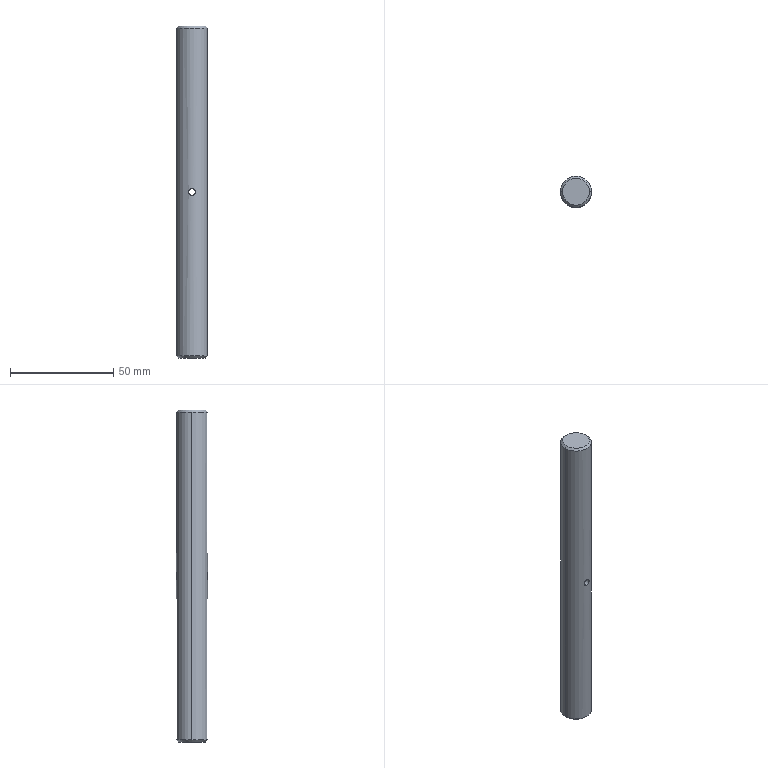Component | SolidWorks | Roller-01-2-1_XT-1-08-2-1 | 1 solid | 10 faces | box 15 x 15 x 160.5 mm | volume 28190 mm3 | cylinder 4 | cone 4 | plane 2 | commonest cylinder face diameters 3.3 x2 15 x2
build123d program:
from build123d import *

# Parameters (mm, degrees)
SKETCH1_R           = 7.5
BOSS_EXTRUDE1_DEPTH = 160.5
CHAMFER1_SIZE       = 1
M4_TAPPED_HOLE1_D   = 3.3


with BuildPart() as part:
    # Sketch1 → Boss-Extrude1 (new body)
    with BuildSketch(Plane.XY):
        Circle(SKETCH1_R)
    extrude(amount=BOSS_EXTRUDE1_DEPTH)

    # Chamfer1
    chamfer1_edges = [part.edges().sort_by_distance(p)[0] for p in [
        (-7.5, 0, 0),
        (-7.5, 0, 160.5),
    ]]
    chamfer(chamfer1_edges, length=CHAMFER1_SIZE)

    # M4 Tapped Hole1 (through all)
    with Locations(Plane(origin=(0, 8.5, 0), x_dir=(1, 0, 0), z_dir=(0, 1, 0))):
        with Locations((0, -80.25)):
            Hole(M4_TAPPED_HOLE1_D / 2)


solid = part.part

# Placed as in the assembly
solid = solid.moved(Location((444.783, 71.385, -153), (0, 0, 0)))
STEP:
#1=CARTESIAN_POINT('',(17.511,2.515,-2.929));
#2=VERTEX_POINT('',#1);
#3=CARTESIAN_POINT('',(17.511,2.515,-2.799));
#4=VERTEX_POINT('',#3);
#5=CARTESIAN_POINT('',(17.511,2.515,-2.929));
#6=CARTESIAN_POINT('',(17.503,2.515,-2.929));
#7=CARTESIAN_POINT('',(17.494,2.516,-2.927));
#8=CARTESIAN_POINT('',(17.482,2.517,-2.923));
#9=CARTESIAN_POINT('',(17.479,2.517,-2.921));
#10=CARTESIAN_POINT('',(17.471,2.518,-2.916));
#11=CARTESIAN_POINT('',(17.468,2.518,-2.913));
#12=CARTESIAN_POINT('',(17.462,2.519,-2.907));
#13=CARTESIAN_POINT('',(17.46,2.52,-2.904));
#14=CARTESIAN_POINT('',(17.455,2.521,-2.897));
#15=CARTESIAN_POINT('',(17.453,2.521,-2.893));
#16=CARTESIAN_POINT('',(17.448,2.522,-2.881));
#17=CARTESIAN_POINT('',(17.446,2.522,-2.873));
#18=CARTESIAN_POINT('',(17.446,2.522,-2.86));
#19=CARTESIAN_POINT('',(17.447,2.522,-2.856));
#20=CARTESIAN_POINT('',(17.448,2.522,-2.847));
#21=CARTESIAN_POINT('',(17.45,2.522,-2.843));
#22=CARTESIAN_POINT('',(17.454,2.521,-2.831));
#23=CARTESIAN_POINT('',(17.459,2.52,-2.824));
#24=CARTESIAN_POINT('',(17.471,2.518,-2.812));
#25=CARTESIAN_POINT('',(17.478,2.517,-2.807));
#26=CARTESIAN_POINT('',(17.49,2.516,-2.803));
#27=CARTESIAN_POINT('',(17.494,2.516,-2.801));
#28=CARTESIAN_POINT('',(17.503,2.515,-2.8));
#29=CARTESIAN_POINT('',(17.507,2.515,-2.799));
#30=CARTESIAN_POINT('',(17.511,2.515,-2.799));
#31=B_SPLINE_CURVE_WITH_KNOTS('',3,(#5,#6,#7,#8,#9,#10,#11,#12,#13,#14,#15,#16,#17,#18,#19,#20,#21,#22,#23,#24,#25,#26,#27,#28,#29,#30),.UNSPECIFIED.,.F.,.F.,(4,2,2,2,2,2,2,2,2,2,2,2,4),(0.005175,0.005821,0.006144,0.006468,0.006791,0.007114,0.007761,0.008084,0.008408,0.009054,0.009701,0.01002,0.01035),.UNSPECIFIED.);
#32=EDGE_CURVE('',#2,#4,#31,.T.);
#33=ORIENTED_EDGE('',*,*,#32,.F.);
#34=CARTESIAN_POINT('',(17.511,3.106,-2.929));
#35=VERTEX_POINT('',#34);
#36=CARTESIAN_POINT('',(17.511,3.145,-2.929));
#37=DIRECTION('',(0.,1.,0.));
#38=VECTOR('',#37,39.37);
#39=LINE('',#36,#38);
#40=EDGE_CURVE('',#2,#35,#39,.T.);
#41=ORIENTED_EDGE('',*,*,#40,.T.);
#42=CARTESIAN_POINT('',(17.511,3.106,-2.799));
#43=VERTEX_POINT('',#42);
#44=CARTESIAN_POINT('',(17.511,3.106,-2.799));
#45=CARTESIAN_POINT('',(17.507,3.106,-2.799));
#46=CARTESIAN_POINT('',(17.503,3.106,-2.8));
#47=CARTESIAN_POINT('',(17.494,3.105,-2.801));
#48=CARTESIAN_POINT('',(17.49,3.105,-2.803));
#49=CARTESIAN_POINT('',(17.482,3.104,-2.806));
#50=CARTESIAN_POINT('',(17.479,3.104,-2.808));
#51=CARTESIAN_POINT('',(17.472,3.103,-2.813));
#52=CARTESIAN_POINT('',(17.468,3.103,-2.815));
#53=CARTESIAN_POINT('',(17.459,3.101,-2.824));
#54=CARTESIAN_POINT('',(17.454,3.1,-2.831));
#55=CARTESIAN_POINT('',(17.448,3.099,-2.847));
#56=CARTESIAN_POINT('',(17.446,3.098,-2.856));
#57=CARTESIAN_POINT('',(17.446,3.098,-2.868));
#58=CARTESIAN_POINT('',(17.447,3.099,-2.873));
#59=CARTESIAN_POINT('',(17.448,3.099,-2.881));
#60=CARTESIAN_POINT('',(17.45,3.099,-2.885));
#61=CARTESIAN_POINT('',(17.454,3.1,-2.897));
#62=CARTESIAN_POINT('',(17.459,3.101,-2.904));
#63=CARTESIAN_POINT('',(17.468,3.103,-2.913));
#64=CARTESIAN_POINT('',(17.472,3.103,-2.916));
#65=CARTESIAN_POINT('',(17.479,3.104,-2.921));
#66=CARTESIAN_POINT('',(17.482,3.104,-2.923));
#67=CARTESIAN_POINT('',(17.49,3.105,-2.926));
#68=CARTESIAN_POINT('',(17.494,3.105,-2.927));
#69=CARTESIAN_POINT('',(17.503,3.106,-2.929));
#70=CARTESIAN_POINT('',(17.507,3.106,-2.929));
#71=CARTESIAN_POINT('',(17.511,3.106,-2.929));
#72=B_SPLINE_CURVE_WITH_KNOTS('',3,(#44,#45,#46,#47,#48,#49,#50,#51,#52,#53,#54,#55,#56,#57,#58,#59,#60,#61,#62,#63,#64,#65,#66,#67,#68,#69,#70,#71),.UNSPECIFIED.,.F.,.F.,(4,2,2,2,2,2,2,2,2,2,2,2,2,4),(0.,0.0003234,0.0006468,0.0009702,0.001294,0.00194,0.002587,0.002911,0.003234,0.003881,0.004204,0.004528,0.004851,0.005175),.UNSPECIFIED.);
#73=EDGE_CURVE('',#43,#35,#72,.T.);
#74=ORIENTED_EDGE('',*,*,#73,.F.);
#75=CARTESIAN_POINT('',(17.511,3.145,-2.799));
#76=DIRECTION('',(0.,1.,0.));
#77=VECTOR('',#76,39.37);
#78=LINE('',#75,#77);
#79=EDGE_CURVE('',#4,#43,#78,.T.);
#80=ORIENTED_EDGE('',*,*,#79,.F.);
#81=EDGE_LOOP('',(#33,#41,#74,#80));
#82=FACE_OUTER_BOUND('',#81,.T.);
#83=CARTESIAN_POINT('',(17.511,3.145,-2.864));
#84=DIRECTION('',(0.,1.,0.));
#85=DIRECTION('',(0.,0.,1.));
#86=AXIS2_PLACEMENT_3D('',#83,#84,#85);
#87=CYLINDRICAL_SURFACE('',#86,0.06496);
#88=ADVANCED_FACE('',(#82),#87,.F.);
#89=CARTESIAN_POINT('',(17.767,2.81,0.2953));
#90=VERTEX_POINT('',#89);
#91=CARTESIAN_POINT('',(17.255,2.81,0.2953));
#92=VERTEX_POINT('',#91);
#93=CARTESIAN_POINT('',(17.511,2.81,0.2953));
#94=DIRECTION('',(0.,0.,1.));
#95=DIRECTION('',(1.,0.,0.));
#96=AXIS2_PLACEMENT_3D('',#93,#94,#95);
#97=CIRCLE('',#96,0.2559);
#98=EDGE_CURVE('',#90,#92,#97,.T.);
#99=ORIENTED_EDGE('',*,*,#98,.F.);
#100=CARTESIAN_POINT('',(17.806,2.81,0.2559));
#101=VERTEX_POINT('',#100);
#102=CARTESIAN_POINT('',(17.767,2.81,0.2953));
#103=DIRECTION('',(0.7071,0.,-0.7071));
#104=VECTOR('',#103,39.37);
#105=LINE('',#102,#104);
#106=EDGE_CURVE('',#90,#101,#105,.T.);
#107=ORIENTED_EDGE('',*,*,#106,.T.);
#108=CARTESIAN_POINT('',(17.216,2.81,0.2559));
#109=VERTEX_POINT('',#108);
#110=CARTESIAN_POINT('',(17.511,2.81,0.2559));
#111=DIRECTION('',(0.,0.,-1.));
#112=DIRECTION('',(1.,0.,0.));
#113=AXIS2_PLACEMENT_3D('',#110,#111,#112);
#114=CIRCLE('',#113,0.2953);
#115=EDGE_CURVE('',#109,#101,#114,.T.);
#116=ORIENTED_EDGE('',*,*,#115,.F.);
#117=CARTESIAN_POINT('',(17.255,2.81,0.2953));
#118=DIRECTION('',(-0.7071,0.,-0.7071));
#119=VECTOR('',#118,39.37);
#120=LINE('',#117,#119);
#121=EDGE_CURVE('',#92,#109,#120,.T.);
#122=ORIENTED_EDGE('',*,*,#121,.F.);
#123=EDGE_LOOP('',(#99,#107,#116,#122));
#124=FACE_OUTER_BOUND('',#123,.T.);
#125=CARTESIAN_POINT('',(17.511,2.81,0.2953));
#126=DIRECTION('',(0.,0.,-1.));
#127=DIRECTION('',(-1.,0.,0.));
#128=AXIS2_PLACEMENT_3D('',#125,#126,#127);
#129=CONICAL_SURFACE('',#128,0.2559,0.7854);
#130=ADVANCED_FACE('',(#124),#129,.T.);
#131=CARTESIAN_POINT('',(17.255,2.81,-6.024));
#132=VERTEX_POINT('',#131);
#133=CARTESIAN_POINT('',(17.767,2.81,-6.024));
#134=VERTEX_POINT('',#133);
#135=CARTESIAN_POINT('',(17.511,2.81,-6.024));
#136=DIRECTION('',(0.,0.,-1.));
#137=DIRECTION('',(1.,0.,0.));
#138=AXIS2_PLACEMENT_3D('',#135,#136,#137);
#139=CIRCLE('',#138,0.2559);
#140=EDGE_CURVE('',#132,#134,#139,.T.);
#141=ORIENTED_EDGE('',*,*,#140,.F.);
#142=CARTESIAN_POINT('',(17.216,2.81,-5.984));
#143=VERTEX_POINT('',#142);
#144=CARTESIAN_POINT('',(17.216,2.81,-5.984));
#145=DIRECTION('',(-0.7071,0.,0.7071));
#146=VECTOR('',#145,39.37);
#147=LINE('',#144,#146);
#148=EDGE_CURVE('',#132,#143,#147,.T.);
#149=ORIENTED_EDGE('',*,*,#148,.T.);
#150=CARTESIAN_POINT('',(17.806,2.81,-5.984));
#151=VERTEX_POINT('',#150);
#152=CARTESIAN_POINT('',(17.511,2.81,-5.984));
#153=DIRECTION('',(0.,0.,1.));
#154=DIRECTION('',(1.,0.,0.));
#155=AXIS2_PLACEMENT_3D('',#152,#153,#154);
#156=CIRCLE('',#155,0.2953);
#157=EDGE_CURVE('',#151,#143,#156,.T.);
#158=ORIENTED_EDGE('',*,*,#157,.F.);
#159=CARTESIAN_POINT('',(17.806,2.81,-5.984));
#160=DIRECTION('',(0.7071,0.,0.7071));
#161=VECTOR('',#160,39.37);
#162=LINE('',#159,#161);
#163=EDGE_CURVE('',#134,#151,#162,.T.);
#164=ORIENTED_EDGE('',*,*,#163,.F.);
#165=EDGE_LOOP('',(#141,#149,#158,#164));
#166=FACE_OUTER_BOUND('',#165,.T.);
#167=CARTESIAN_POINT('',(17.511,2.81,-5.984));
#168=DIRECTION('',(0.,0.,1.));
#169=DIRECTION('',(1.,0.,0.));
#170=AXIS2_PLACEMENT_3D('',#167,#168,#169);
#171=CONICAL_SURFACE('',#170,0.2953,0.7854);
#172=ADVANCED_FACE('',(#166),#171,.T.);
#173=ORIENTED_EDGE('',*,*,#73,.T.);
#174=CARTESIAN_POINT('',(17.511,3.106,-2.929));
#175=CARTESIAN_POINT('',(17.52,3.106,-2.929));
#176=CARTESIAN_POINT('',(17.528,3.105,-2.927));
#177=CARTESIAN_POINT('',(17.54,3.104,-2.923));
#178=CARTESIAN_POINT('',(17.544,3.104,-2.921));
#179=CARTESIAN_POINT('',(17.551,3.103,-2.916));
#180=CARTESIAN_POINT('',(17.554,3.103,-2.913));
#181=CARTESIAN_POINT('',(17.56,3.102,-2.907));
#182=CARTESIAN_POINT('',(17.563,3.101,-2.904));
#183=CARTESIAN_POINT('',(17.567,3.1,-2.897));
#184=CARTESIAN_POINT('',(17.569,3.1,-2.893));
#185=CARTESIAN_POINT('',(17.574,3.099,-2.881));
#186=CARTESIAN_POINT('',(17.576,3.098,-2.873));
#187=CARTESIAN_POINT('',(17.576,3.098,-2.86));
#188=CARTESIAN_POINT('',(17.576,3.099,-2.856));
#189=CARTESIAN_POINT('',(17.574,3.099,-2.847));
#190=CARTESIAN_POINT('',(17.573,3.099,-2.843));
#191=CARTESIAN_POINT('',(17.568,3.1,-2.831));
#192=CARTESIAN_POINT('',(17.563,3.101,-2.824));
#193=CARTESIAN_POINT('',(17.551,3.103,-2.812));
#194=CARTESIAN_POINT('',(17.544,3.104,-2.807));
#195=CARTESIAN_POINT('',(17.532,3.105,-2.803));
#196=CARTESIAN_POINT('',(17.528,3.105,-2.801));
#197=CARTESIAN_POINT('',(17.52,3.106,-2.8));
#198=CARTESIAN_POINT('',(17.515,3.106,-2.799));
#199=CARTESIAN_POINT('',(17.511,3.106,-2.799));
#200=B_SPLINE_CURVE_WITH_KNOTS('',3,(#174,#175,#176,#177,#178,#179,#180,#181,#182,#183,#184,#185,#186,#187,#188,#189,#190,#191,#192,#193,#194,#195,#196,#197,#198,#199),.UNSPECIFIED.,.F.,.F.,(4,2,2,2,2,2,2,2,2,2,2,2,4),(0.005175,0.005821,0.006144,0.006468,0.006791,0.007114,0.007761,0.008084,0.008408,0.009054,0.009701,0.01002,0.01035),.UNSPECIFIED.);
#201=EDGE_CURVE('',#35,#43,#200,.T.);
#202=ORIENTED_EDGE('',*,*,#201,.T.);
#203=EDGE_LOOP('',(#173,#202));
#204=FACE_BOUND('',#203,.T.);
#205=ORIENTED_EDGE('',*,*,#115,.T.);
#206=CARTESIAN_POINT('',(17.806,2.81,0.2953));
#207=DIRECTION('',(0.,0.,-1.));
#208=VECTOR('',#207,39.37);
#209=LINE('',#206,#208);
#210=EDGE_CURVE('',#101,#151,#209,.T.);
#211=ORIENTED_EDGE('',*,*,#210,.T.);
#212=ORIENTED_EDGE('',*,*,#157,.T.);
#213=CARTESIAN_POINT('',(17.216,2.81,0.2953));
#214=DIRECTION('',(0.,0.,-1.));
#215=VECTOR('',#214,39.37);
#216=LINE('',#213,#215);
#217=EDGE_CURVE('',#109,#143,#216,.T.);
#218=ORIENTED_EDGE('',*,*,#217,.F.);
#219=EDGE_LOOP('',(#205,#211,#212,#218));
#220=FACE_OUTER_BOUND('',#219,.T.);
#221=CARTESIAN_POINT('',(17.511,2.81,0.2953));
#222=DIRECTION('',(0.,0.,-1.));
#223=DIRECTION('',(-1.,0.,0.));
#224=AXIS2_PLACEMENT_3D('',#221,#222,#223);
#225=CYLINDRICAL_SURFACE('',#224,0.2953);
#226=ADVANCED_FACE('',(#204,#220),#225,.T.);
#227=ORIENTED_EDGE('',*,*,#210,.F.);
#228=CARTESIAN_POINT('',(17.511,2.81,0.2559));
#229=DIRECTION('',(0.,0.,-1.));
#230=DIRECTION('',(1.,0.,0.));
#231=AXIS2_PLACEMENT_3D('',#228,#229,#230);
#232=CIRCLE('',#231,0.2953);
#233=EDGE_CURVE('',#101,#109,#232,.T.);
#234=ORIENTED_EDGE('',*,*,#233,.T.);
#235=ORIENTED_EDGE('',*,*,#217,.T.);
#236=CARTESIAN_POINT('',(17.511,2.81,-5.984));
#237=DIRECTION('',(0.,0.,1.));
#238=DIRECTION('',(1.,0.,0.));
#239=AXIS2_PLACEMENT_3D('',#236,#237,#238);
#240=CIRCLE('',#239,0.2953);
#241=EDGE_CURVE('',#143,#151,#240,.T.);
#242=ORIENTED_EDGE('',*,*,#241,.T.);
#243=EDGE_LOOP('',(#227,#234,#235,#242));
#244=FACE_OUTER_BOUND('',#243,.T.);
#245=CARTESIAN_POINT('',(17.511,2.515,-2.799));
#246=CARTESIAN_POINT('',(17.515,2.515,-2.799));
#247=CARTESIAN_POINT('',(17.52,2.515,-2.8));
#248=CARTESIAN_POINT('',(17.528,2.516,-2.801));
#249=CARTESIAN_POINT('',(17.532,2.516,-2.803));
#250=CARTESIAN_POINT('',(17.54,2.517,-2.806));
#251=CARTESIAN_POINT('',(17.544,2.517,-2.808));
#252=CARTESIAN_POINT('',(17.551,2.518,-2.813));
#253=CARTESIAN_POINT('',(17.554,2.518,-2.815));
#254=CARTESIAN_POINT('',(17.563,2.52,-2.824));
#255=CARTESIAN_POINT('',(17.568,2.521,-2.831));
#256=CARTESIAN_POINT('',(17.574,2.522,-2.847));
#257=CARTESIAN_POINT('',(17.576,2.522,-2.856));
#258=CARTESIAN_POINT('',(17.576,2.522,-2.868));
#259=CARTESIAN_POINT('',(17.576,2.522,-2.873));
#260=CARTESIAN_POINT('',(17.574,2.522,-2.881));
#261=CARTESIAN_POINT('',(17.573,2.522,-2.885));
#262=CARTESIAN_POINT('',(17.568,2.521,-2.897));
#263=CARTESIAN_POINT('',(17.563,2.52,-2.904));
#264=CARTESIAN_POINT('',(17.554,2.518,-2.913));
#265=CARTESIAN_POINT('',(17.551,2.518,-2.916));
#266=CARTESIAN_POINT('',(17.544,2.517,-2.921));
#267=CARTESIAN_POINT('',(17.54,2.517,-2.923));
#268=CARTESIAN_POINT('',(17.532,2.516,-2.926));
#269=CARTESIAN_POINT('',(17.528,2.516,-2.927));
#270=CARTESIAN_POINT('',(17.52,2.515,-2.929));
#271=CARTESIAN_POINT('',(17.515,2.515,-2.929));
#272=CARTESIAN_POINT('',(17.511,2.515,-2.929));
#273=B_SPLINE_CURVE_WITH_KNOTS('',3,(#245,#246,#247,#248,#249,#250,#251,#252,#253,#254,#255,#256,#257,#258,#259,#260,#261,#262,#263,#264,#265,#266,#267,#268,#269,#270,#271,#272),.UNSPECIFIED.,.F.,.F.,(4,2,2,2,2,2,2,2,2,2,2,2,2,4),(0.,0.0003234,0.0006468,0.0009702,0.001294,0.00194,0.002587,0.002911,0.003234,0.003881,0.004204,0.004528,0.004851,0.005175),.UNSPECIFIED.);
#274=EDGE_CURVE('',#4,#2,#273,.T.);
#275=ORIENTED_EDGE('',*,*,#274,.T.);
#276=ORIENTED_EDGE('',*,*,#32,.T.);
#277=EDGE_LOOP('',(#275,#276));
#278=FACE_BOUND('',#277,.T.);
#279=CARTESIAN_POINT('',(17.511,2.81,0.2953));
#280=DIRECTION('',(0.,0.,-1.));
#281=DIRECTION('',(-1.,0.,0.));
#282=AXIS2_PLACEMENT_3D('',#279,#280,#281);
#283=CYLINDRICAL_SURFACE('',#282,0.2953);
#284=ADVANCED_FACE('',(#244,#278),#283,.T.);
#285=CARTESIAN_POINT('',(17.511,2.81,0.2953));
#286=DIRECTION('',(0.,0.,1.));
#287=DIRECTION('',(1.,0.,0.));
#288=AXIS2_PLACEMENT_3D('',#285,#286,#287);
#289=CIRCLE('',#288,0.2559);
#290=EDGE_CURVE('',#92,#90,#289,.T.);
#291=ORIENTED_EDGE('',*,*,#290,.T.);
#292=ORIENTED_EDGE('',*,*,#98,.T.);
#293=EDGE_LOOP('',(#291,#292));
#294=FACE_OUTER_BOUND('',#293,.T.);
#295=CARTESIAN_POINT('',(17.511,2.81,0.2953));
#296=DIRECTION('',(0.,0.,1.));
#297=DIRECTION('',(1.,0.,0.));
#298=AXIS2_PLACEMENT_3D('',#295,#296,#297);
#299=PLANE('',#298);
#300=ADVANCED_FACE('',(#294),#299,.T.);
#301=CARTESIAN_POINT('',(17.511,2.81,-6.024));
#302=DIRECTION('',(0.,0.,-1.));
#303=DIRECTION('',(1.,0.,0.));
#304=AXIS2_PLACEMENT_3D('',#301,#302,#303);
#305=CIRCLE('',#304,0.2559);
#306=EDGE_CURVE('',#134,#132,#305,.T.);
#307=ORIENTED_EDGE('',*,*,#306,.T.);
#308=ORIENTED_EDGE('',*,*,#140,.T.);
#309=EDGE_LOOP('',(#307,#308));
#310=FACE_OUTER_BOUND('',#309,.T.);
#311=CARTESIAN_POINT('',(17.511,2.81,-6.024));
#312=DIRECTION('',(0.,0.,1.));
#313=DIRECTION('',(1.,0.,0.));
#314=AXIS2_PLACEMENT_3D('',#311,#312,#313);
#315=PLANE('',#314);
#316=ADVANCED_FACE('',(#310),#315,.F.);
#317=ORIENTED_EDGE('',*,*,#148,.F.);
#318=ORIENTED_EDGE('',*,*,#306,.F.);
#319=ORIENTED_EDGE('',*,*,#163,.T.);
#320=ORIENTED_EDGE('',*,*,#241,.F.);
#321=EDGE_LOOP('',(#317,#318,#319,#320));
#322=FACE_OUTER_BOUND('',#321,.T.);
#323=CARTESIAN_POINT('',(17.511,2.81,-5.984));
#324=DIRECTION('',(0.,0.,1.));
#325=DIRECTION('',(1.,0.,0.));
#326=AXIS2_PLACEMENT_3D('',#323,#324,#325);
#327=CONICAL_SURFACE('',#326,0.2953,0.7854);
#328=ADVANCED_FACE('',(#322),#327,.T.);
#329=ORIENTED_EDGE('',*,*,#106,.F.);
#330=ORIENTED_EDGE('',*,*,#290,.F.);
#331=ORIENTED_EDGE('',*,*,#121,.T.);
#332=ORIENTED_EDGE('',*,*,#233,.F.);
#333=EDGE_LOOP('',(#329,#330,#331,#332));
#334=FACE_OUTER_BOUND('',#333,.T.);
#335=CARTESIAN_POINT('',(17.511,2.81,0.2953));
#336=DIRECTION('',(0.,0.,-1.));
#337=DIRECTION('',(-1.,0.,0.));
#338=AXIS2_PLACEMENT_3D('',#335,#336,#337);
#339=CONICAL_SURFACE('',#338,0.2559,0.7854);
#340=ADVANCED_FACE('',(#334),#339,.T.);
#341=ORIENTED_EDGE('',*,*,#40,.F.);
#342=ORIENTED_EDGE('',*,*,#274,.F.);
#343=ORIENTED_EDGE('',*,*,#79,.T.);
#344=ORIENTED_EDGE('',*,*,#201,.F.);
#345=EDGE_LOOP('',(#341,#342,#343,#344));
#346=FACE_OUTER_BOUND('',#345,.T.);
#347=CARTESIAN_POINT('',(17.511,3.145,-2.864));
#348=DIRECTION('',(0.,1.,0.));
#349=DIRECTION('',(0.,0.,1.));
#350=AXIS2_PLACEMENT_3D('',#347,#348,#349);
#351=CYLINDRICAL_SURFACE('',#350,0.06496);
#352=ADVANCED_FACE('',(#346),#351,.F.);
#353=CLOSED_SHELL('',(#88,#130,#172,#226,#284,#300,#316,#328,#340,#352));
#354=MANIFOLD_SOLID_BREP('',#353);
#355=CARTESIAN_POINT('',(0.,0.,0.));
#356=DIRECTION('',(0.,0.,1.));
#357=DIRECTION('',(1.,0.,0.));
#358=AXIS2_PLACEMENT_3D('',#355,#356,#357);
#359=(LENGTH_UNIT()NAMED_UNIT(*)SI_UNIT($,.METRE.));
#360=LENGTH_MEASURE_WITH_UNIT(LENGTH_MEASURE(0.0254),#359);
#361=DIMENSIONAL_EXPONENTS(1.,0.,0.,0.,0.,0.,0.);
#362=(CONVERSION_BASED_UNIT('',#360)LENGTH_UNIT()NAMED_UNIT(#361));
#363=UNCERTAINTY_MEASURE_WITH_UNIT(LENGTH_MEASURE(0.00001),#362,'','');
#364=(NAMED_UNIT(*)PLANE_ANGLE_UNIT()SI_UNIT($,.RADIAN.));
#365=(NAMED_UNIT(*)SI_UNIT($,.STERADIAN.)SOLID_ANGLE_UNIT());
#366=(GEOMETRIC_REPRESENTATION_CONTEXT(3)GLOBAL_UNCERTAINTY_ASSIGNED_CONTEXT((#363))GLOBAL_UNIT_ASSIGNED_CONTEXT((#362,#364,#365))REPRESENTATION_CONTEXT('',''));
#367=ADVANCED_BREP_SHAPE_REPRESENTATION('',(#354,#358),#366);
#368=COLOUR_RGB('',0.7922,0.8196,0.9333);
#369=FILL_AREA_STYLE_COLOUR('',#368);
#370=FILL_AREA_STYLE('',(#369));
#371=SURFACE_STYLE_FILL_AREA(#370);
#372=SURFACE_SIDE_STYLE('',(#371));
#373=SURFACE_STYLE_USAGE(.BOTH.,#372);
#374=PRESENTATION_STYLE_ASSIGNMENT((#373));
#375=STYLED_ITEM('',(#374),#354);
#376=PRESENTATION_LAYER_ASSIGNMENT('','',(#375));
#377=(LENGTH_UNIT()NAMED_UNIT(*)SI_UNIT($,.METRE.));
#378=LENGTH_MEASURE_WITH_UNIT(LENGTH_MEASURE(0.0254),#377);
#379=DIMENSIONAL_EXPONENTS(1.,0.,0.,0.,0.,0.,0.);
#380=(CONVERSION_BASED_UNIT('',#378)LENGTH_UNIT()NAMED_UNIT(#379));
#381=UNCERTAINTY_MEASURE_WITH_UNIT(LENGTH_MEASURE(0.00001),#380,'','');
#382=(NAMED_UNIT(*)PLANE_ANGLE_UNIT()SI_UNIT($,.RADIAN.));
#383=(NAMED_UNIT(*)SI_UNIT($,.STERADIAN.)SOLID_ANGLE_UNIT());
#384=(GEOMETRIC_REPRESENTATION_CONTEXT(3)GLOBAL_UNCERTAINTY_ASSIGNED_CONTEXT((#381))GLOBAL_UNIT_ASSIGNED_CONTEXT((#380,#382,#383))REPRESENTATION_CONTEXT('',''));
#385=MECHANICAL_DESIGN_GEOMETRIC_PRESENTATION_REPRESENTATION('',(#375),#384);